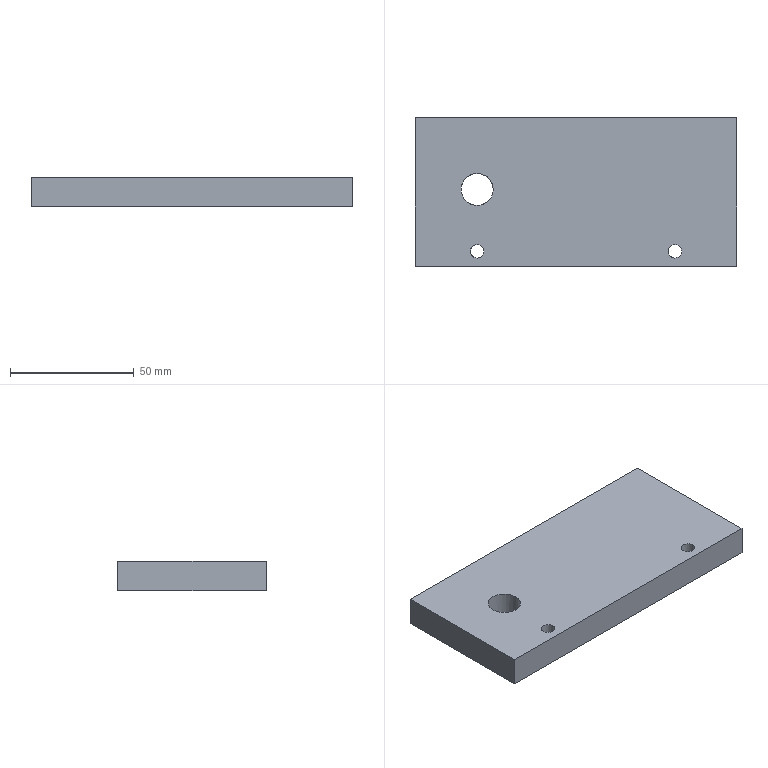Component | NX | Root-owned geometry | 1 solid | 13 faces | box 130 x 60 x 12 mm | volume 90813 mm3 | plane 8 | cylinder 5 | commonest cylinder face diameters 5.5 x2 10 x2 13 x1
STEP:
#1=CARTESIAN_POINT('',(0.,0.,0.));
#2=DIRECTION('',(0.,0.,1.));
#3=DIRECTION('',(1.,0.,0.));
#4=AXIS2_PLACEMENT_3D('',#1,#2,#3);
#5=CARTESIAN_POINT('',(40.,-21.25,12.));
#6=VERTEX_POINT('',#5);
#7=CARTESIAN_POINT('',(40.,-24.,12.));
#8=DIRECTION('',(0.,0.,-1.));
#9=DIRECTION('',(0.,1.,0.));
#10=AXIS2_PLACEMENT_3D('',#7,#8,#9);
#11=CIRCLE('',#10,2.75);
#12=CARTESIAN_POINT('',(40.,-24.,-20.));
#13=DIRECTION('',(0.,0.,1.));
#14=DIRECTION('',(1.,0.,0.));
#15=AXIS2_PLACEMENT_3D('',#12,#13,#14);
#16=CYLINDRICAL_SURFACE('',#15,2.75);
#17=CARTESIAN_POINT('',(7.854,32.));
#18=DIRECTION('',(-1.,0.));
#19=VECTOR('',#18,1.);
#20=LINE('',#17,#19);
#21=(GEOMETRIC_REPRESENTATION_CONTEXT(2)PARAMETRIC_REPRESENTATION_CONTEXT()REPRESENTATION_CONTEXT('',''));
#22=DEFINITIONAL_REPRESENTATION('',(#20),#21);
#23=PCURVE('',#16,#22);
#24=CARTESIAN_POINT('',(0.,0.,12.));
#25=DIRECTION('',(0.,0.,1.));
#26=DIRECTION('',(1.,0.,0.));
#27=AXIS2_PLACEMENT_3D('',#24,#25,#26);
#28=PLANE('',#27);
#29=CARTESIAN_POINT('',(40.,-21.25));
#30=CARTESIAN_POINT('',(44.763,-21.25));
#31=CARTESIAN_POINT('',(42.382,-25.375));
#32=CARTESIAN_POINT('',(40.,-29.5));
#33=CARTESIAN_POINT('',(37.618,-25.375));
#34=CARTESIAN_POINT('',(35.237,-21.25));
#35=CARTESIAN_POINT('',(40.,-21.25));
#36=(BOUNDED_CURVE()B_SPLINE_CURVE(2,(#29,#30,#31,#32,#33,#34,#35),.UNSPECIFIED.,.T.,.F.)B_SPLINE_CURVE_WITH_KNOTS((1,2,2,2,2,1),(-2.094,0.,2.094,4.189,6.283,8.378),.UNSPECIFIED.)CURVE()GEOMETRIC_REPRESENTATION_ITEM()RATIONAL_B_SPLINE_CURVE((1.,0.5,1.,0.5,1.,0.5,1.))REPRESENTATION_ITEM(''));
#37=(GEOMETRIC_REPRESENTATION_CONTEXT(2)PARAMETRIC_REPRESENTATION_CONTEXT()REPRESENTATION_CONTEXT('',''));
#38=DEFINITIONAL_REPRESENTATION('',(#36),#37);
#39=PCURVE('',#28,#38);
#40=SURFACE_CURVE('',#11,(#23,#39),.PCURVE_S1.);
#41=EDGE_CURVE('',#6,#6,#40,.T.);
#42=ORIENTED_EDGE('',*,*,#41,.T.);
#43=CARTESIAN_POINT('',(40.,-21.25,5.7));
#44=VERTEX_POINT('',#43);
#45=CARTESIAN_POINT('',(40.,-21.25,5.7));
#46=CARTESIAN_POINT('',(40.,-21.25,12.));
#47=B_SPLINE_CURVE_WITH_KNOTS('',1,(#45,#46),.UNSPECIFIED.,.F.,.F.,(2,2),(25.7,32.),.PIECEWISE_BEZIER_KNOTS.);
#48=CARTESIAN_POINT('',(1.571,0.));
#49=DIRECTION('',(0.,1.));
#50=VECTOR('',#49,1.);
#51=LINE('',#48,#50);
#52=(GEOMETRIC_REPRESENTATION_CONTEXT(2)PARAMETRIC_REPRESENTATION_CONTEXT()REPRESENTATION_CONTEXT('',''));
#53=DEFINITIONAL_REPRESENTATION('',(#51),#52);
#54=PCURVE('',#16,#53);
#55=CARTESIAN_POINT('',(7.854,0.));
#56=DIRECTION('',(0.,1.));
#57=VECTOR('',#56,1.);
#58=LINE('',#55,#57);
#59=(GEOMETRIC_REPRESENTATION_CONTEXT(2)PARAMETRIC_REPRESENTATION_CONTEXT()REPRESENTATION_CONTEXT('',''));
#60=DEFINITIONAL_REPRESENTATION('',(#58),#59);
#61=PCURVE('',#16,#60);
#62=SEAM_CURVE('',#47,(#54,#61),.PCURVE_S1.);
#63=EDGE_CURVE('',#44,#6,#62,.T.);
#64=ORIENTED_EDGE('',*,*,#63,.F.);
#65=CARTESIAN_POINT('',(37.25,-24.,5.7));
#66=VERTEX_POINT('',#65);
#67=CARTESIAN_POINT('',(40.,-24.,5.7));
#68=DIRECTION('',(0.,0.,-1.));
#69=DIRECTION('',(-1.,0.,0.));
#70=AXIS2_PLACEMENT_3D('',#67,#68,#69);
#71=CIRCLE('',#70,2.75);
#72=CARTESIAN_POINT('',(3.142,25.7));
#73=DIRECTION('',(-1.,0.));
#74=VECTOR('',#73,1.);
#75=LINE('',#72,#74);
#76=(GEOMETRIC_REPRESENTATION_CONTEXT(2)PARAMETRIC_REPRESENTATION_CONTEXT()REPRESENTATION_CONTEXT('',''));
#77=DEFINITIONAL_REPRESENTATION('',(#75),#76);
#78=PCURVE('',#16,#77);
#79=CARTESIAN_POINT('',(40.,-24.,5.7));
#80=DIRECTION('',(0.,0.,-1.));
#81=DIRECTION('',(-1.,0.,0.));
#82=AXIS2_PLACEMENT_3D('',#79,#80,#81);
#83=PLANE('',#82);
#84=CARTESIAN_POINT('',(0.,0.));
#85=DIRECTION('',(1.,0.));
#86=AXIS2_PLACEMENT_2D('',#84,#85);
#87=CIRCLE('',#86,2.75);
#88=(GEOMETRIC_REPRESENTATION_CONTEXT(2)PARAMETRIC_REPRESENTATION_CONTEXT()REPRESENTATION_CONTEXT('',''));
#89=DEFINITIONAL_REPRESENTATION('',(#87),#88);
#90=PCURVE('',#83,#89);
#91=SURFACE_CURVE('',#71,(#78,#90),.PCURVE_S1.);
#92=EDGE_CURVE('',#66,#44,#91,.T.);
#93=ORIENTED_EDGE('',*,*,#92,.F.);
#94=CARTESIAN_POINT('',(40.,-24.,5.7));
#95=DIRECTION('',(0.,0.,-1.));
#96=DIRECTION('',(-1.,0.,0.));
#97=AXIS2_PLACEMENT_3D('',#94,#95,#96);
#98=CIRCLE('',#97,2.75);
#99=CARTESIAN_POINT('',(9.425,25.7));
#100=DIRECTION('',(-1.,0.));
#101=VECTOR('',#100,1.);
#102=LINE('',#99,#101);
#103=(GEOMETRIC_REPRESENTATION_CONTEXT(2)PARAMETRIC_REPRESENTATION_CONTEXT()REPRESENTATION_CONTEXT('',''));
#104=DEFINITIONAL_REPRESENTATION('',(#102),#103);
#105=PCURVE('',#16,#104);
#106=CARTESIAN_POINT('',(0.,0.));
#107=DIRECTION('',(1.,0.));
#108=AXIS2_PLACEMENT_2D('',#106,#107);
#109=CIRCLE('',#108,2.75);
#110=(GEOMETRIC_REPRESENTATION_CONTEXT(2)PARAMETRIC_REPRESENTATION_CONTEXT()REPRESENTATION_CONTEXT('',''));
#111=DEFINITIONAL_REPRESENTATION('',(#109),#110);
#112=PCURVE('',#83,#111);
#113=SURFACE_CURVE('',#98,(#105,#112),.PCURVE_S1.);
#114=EDGE_CURVE('',#44,#66,#113,.T.);
#115=ORIENTED_EDGE('',*,*,#114,.F.);
#116=ORIENTED_EDGE('',*,*,#63,.T.);
#117=EDGE_LOOP('',(#42,#64,#93,#115,#116));
#118=FACE_BOUND('',#117,.F.);
#119=ADVANCED_FACE('',(#118),#16,.F.);
#120=CARTESIAN_POINT('',(-40.,-21.25,12.));
#121=VERTEX_POINT('',#120);
#122=CARTESIAN_POINT('',(-40.,-24.,12.));
#123=DIRECTION('',(0.,0.,-1.));
#124=DIRECTION('',(0.,1.,0.));
#125=AXIS2_PLACEMENT_3D('',#122,#123,#124);
#126=CIRCLE('',#125,2.75);
#127=CARTESIAN_POINT('',(-40.,-24.,-20.));
#128=DIRECTION('',(0.,0.,1.));
#129=DIRECTION('',(1.,0.,0.));
#130=AXIS2_PLACEMENT_3D('',#127,#128,#129);
#131=CYLINDRICAL_SURFACE('',#130,2.75);
#132=CARTESIAN_POINT('',(7.854,32.));
#133=DIRECTION('',(-1.,0.));
#134=VECTOR('',#133,1.);
#135=LINE('',#132,#134);
#136=(GEOMETRIC_REPRESENTATION_CONTEXT(2)PARAMETRIC_REPRESENTATION_CONTEXT()REPRESENTATION_CONTEXT('',''));
#137=DEFINITIONAL_REPRESENTATION('',(#135),#136);
#138=PCURVE('',#131,#137);
#139=CARTESIAN_POINT('',(-40.,-21.25));
#140=CARTESIAN_POINT('',(-35.237,-21.25));
#141=CARTESIAN_POINT('',(-37.618,-25.375));
#142=CARTESIAN_POINT('',(-40.,-29.5));
#143=CARTESIAN_POINT('',(-42.382,-25.375));
#144=CARTESIAN_POINT('',(-44.763,-21.25));
#145=CARTESIAN_POINT('',(-40.,-21.25));
#146=(BOUNDED_CURVE()B_SPLINE_CURVE(2,(#139,#140,#141,#142,#143,#144,#145),.UNSPECIFIED.,.T.,.F.)B_SPLINE_CURVE_WITH_KNOTS((1,2,2,2,2,1),(-2.094,0.,2.094,4.189,6.283,8.378),.UNSPECIFIED.)CURVE()GEOMETRIC_REPRESENTATION_ITEM()RATIONAL_B_SPLINE_CURVE((1.,0.5,1.,0.5,1.,0.5,1.))REPRESENTATION_ITEM(''));
#147=(GEOMETRIC_REPRESENTATION_CONTEXT(2)PARAMETRIC_REPRESENTATION_CONTEXT()REPRESENTATION_CONTEXT('',''));
#148=DEFINITIONAL_REPRESENTATION('',(#146),#147);
#149=PCURVE('',#28,#148);
#150=SURFACE_CURVE('',#126,(#138,#149),.PCURVE_S1.);
#151=EDGE_CURVE('',#121,#121,#150,.T.);
#152=ORIENTED_EDGE('',*,*,#151,.T.);
#153=CARTESIAN_POINT('',(-40.,-21.25,5.7));
#154=VERTEX_POINT('',#153);
#155=CARTESIAN_POINT('',(-40.,-21.25,5.7));
#156=CARTESIAN_POINT('',(-40.,-21.25,12.));
#157=B_SPLINE_CURVE_WITH_KNOTS('',1,(#155,#156),.UNSPECIFIED.,.F.,.F.,(2,2),(25.7,32.),.PIECEWISE_BEZIER_KNOTS.);
#158=CARTESIAN_POINT('',(1.571,0.));
#159=DIRECTION('',(0.,1.));
#160=VECTOR('',#159,1.);
#161=LINE('',#158,#160);
#162=(GEOMETRIC_REPRESENTATION_CONTEXT(2)PARAMETRIC_REPRESENTATION_CONTEXT()REPRESENTATION_CONTEXT('',''));
#163=DEFINITIONAL_REPRESENTATION('',(#161),#162);
#164=PCURVE('',#131,#163);
#165=CARTESIAN_POINT('',(7.854,0.));
#166=DIRECTION('',(0.,1.));
#167=VECTOR('',#166,1.);
#168=LINE('',#165,#167);
#169=(GEOMETRIC_REPRESENTATION_CONTEXT(2)PARAMETRIC_REPRESENTATION_CONTEXT()REPRESENTATION_CONTEXT('',''));
#170=DEFINITIONAL_REPRESENTATION('',(#168),#169);
#171=PCURVE('',#131,#170);
#172=SEAM_CURVE('',#157,(#164,#171),.PCURVE_S1.);
#173=EDGE_CURVE('',#154,#121,#172,.T.);
#174=ORIENTED_EDGE('',*,*,#173,.F.);
#175=CARTESIAN_POINT('',(-42.75,-24.,5.7));
#176=VERTEX_POINT('',#175);
#177=CARTESIAN_POINT('',(-40.,-24.,5.7));
#178=DIRECTION('',(0.,0.,-1.));
#179=DIRECTION('',(-1.,0.,0.));
#180=AXIS2_PLACEMENT_3D('',#177,#178,#179);
#181=CIRCLE('',#180,2.75);
#182=CARTESIAN_POINT('',(3.142,25.7));
#183=DIRECTION('',(-1.,0.));
#184=VECTOR('',#183,1.);
#185=LINE('',#182,#184);
#186=(GEOMETRIC_REPRESENTATION_CONTEXT(2)PARAMETRIC_REPRESENTATION_CONTEXT()REPRESENTATION_CONTEXT('',''));
#187=DEFINITIONAL_REPRESENTATION('',(#185),#186);
#188=PCURVE('',#131,#187);
#189=CARTESIAN_POINT('',(-40.,-24.,5.7));
#190=DIRECTION('',(0.,0.,-1.));
#191=DIRECTION('',(-1.,0.,0.));
#192=AXIS2_PLACEMENT_3D('',#189,#190,#191);
#193=PLANE('',#192);
#194=CARTESIAN_POINT('',(0.,0.));
#195=DIRECTION('',(1.,0.));
#196=AXIS2_PLACEMENT_2D('',#194,#195);
#197=CIRCLE('',#196,2.75);
#198=(GEOMETRIC_REPRESENTATION_CONTEXT(2)PARAMETRIC_REPRESENTATION_CONTEXT()REPRESENTATION_CONTEXT('',''));
#199=DEFINITIONAL_REPRESENTATION('',(#197),#198);
#200=PCURVE('',#193,#199);
#201=SURFACE_CURVE('',#181,(#188,#200),.PCURVE_S1.);
#202=EDGE_CURVE('',#176,#154,#201,.T.);
#203=ORIENTED_EDGE('',*,*,#202,.F.);
#204=CARTESIAN_POINT('',(-40.,-24.,5.7));
#205=DIRECTION('',(0.,0.,-1.));
#206=DIRECTION('',(-1.,0.,0.));
#207=AXIS2_PLACEMENT_3D('',#204,#205,#206);
#208=CIRCLE('',#207,2.75);
#209=CARTESIAN_POINT('',(9.425,25.7));
#210=DIRECTION('',(-1.,0.));
#211=VECTOR('',#210,1.);
#212=LINE('',#209,#211);
#213=(GEOMETRIC_REPRESENTATION_CONTEXT(2)PARAMETRIC_REPRESENTATION_CONTEXT()REPRESENTATION_CONTEXT('',''));
#214=DEFINITIONAL_REPRESENTATION('',(#212),#213);
#215=PCURVE('',#131,#214);
#216=CARTESIAN_POINT('',(0.,0.));
#217=DIRECTION('',(1.,0.));
#218=AXIS2_PLACEMENT_2D('',#216,#217);
#219=CIRCLE('',#218,2.75);
#220=(GEOMETRIC_REPRESENTATION_CONTEXT(2)PARAMETRIC_REPRESENTATION_CONTEXT()REPRESENTATION_CONTEXT('',''));
#221=DEFINITIONAL_REPRESENTATION('',(#219),#220);
#222=PCURVE('',#193,#221);
#223=SURFACE_CURVE('',#208,(#215,#222),.PCURVE_S1.);
#224=EDGE_CURVE('',#154,#176,#223,.T.);
#225=ORIENTED_EDGE('',*,*,#224,.F.);
#226=ORIENTED_EDGE('',*,*,#173,.T.);
#227=EDGE_LOOP('',(#152,#174,#203,#225,#226));
#228=FACE_BOUND('',#227,.F.);
#229=ADVANCED_FACE('',(#228),#131,.F.);
#230=CARTESIAN_POINT('',(-65.,-30.,0.));
#231=VERTEX_POINT('',#230);
#232=CARTESIAN_POINT('',(65.,-30.,0.));
#233=VERTEX_POINT('',#232);
#234=CARTESIAN_POINT('',(-65.,-30.,0.));
#235=DIRECTION('',(1.,0.,0.));
#236=VECTOR('',#235,1.);
#237=LINE('',#234,#236);
#238=CARTESIAN_POINT('',(-65.,-30.,12.));
#239=DIRECTION('',(-0.,1.,0.));
#240=DIRECTION('',(-1.,-0.,0.));
#241=AXIS2_PLACEMENT_3D('',#238,#239,#240);
#242=PLANE('',#241);
#243=CARTESIAN_POINT('',(0.,-12.));
#244=DIRECTION('',(-1.,0.));
#245=VECTOR('',#244,1.);
#246=LINE('',#243,#245);
#247=(GEOMETRIC_REPRESENTATION_CONTEXT(2)PARAMETRIC_REPRESENTATION_CONTEXT()REPRESENTATION_CONTEXT('',''));
#248=DEFINITIONAL_REPRESENTATION('',(#246),#247);
#249=PCURVE('',#242,#248);
#250=CARTESIAN_POINT('',(0.,0.,0.));
#251=DIRECTION('',(0.,0.,1.));
#252=DIRECTION('',(1.,0.,0.));
#253=AXIS2_PLACEMENT_3D('',#250,#251,#252);
#254=PLANE('',#253);
#255=CARTESIAN_POINT('',(-65.,-30.));
#256=DIRECTION('',(1.,0.));
#257=VECTOR('',#256,1.);
#258=LINE('',#255,#257);
#259=(GEOMETRIC_REPRESENTATION_CONTEXT(2)PARAMETRIC_REPRESENTATION_CONTEXT()REPRESENTATION_CONTEXT('',''));
#260=DEFINITIONAL_REPRESENTATION('',(#258),#259);
#261=PCURVE('',#254,#260);
#262=SURFACE_CURVE('',#237,(#249,#261),.PCURVE_S1.);
#263=EDGE_CURVE('',#231,#233,#262,.T.);
#264=ORIENTED_EDGE('',*,*,#263,.T.);
#265=CARTESIAN_POINT('',(65.,-30.,12.));
#266=VERTEX_POINT('',#265);
#267=CARTESIAN_POINT('',(65.,-30.,12.));
#268=DIRECTION('',(0.,0.,-1.));
#269=VECTOR('',#268,1.);
#270=LINE('',#267,#269);
#271=CARTESIAN_POINT('',(-130.,0.));
#272=DIRECTION('',(0.,-1.));
#273=VECTOR('',#272,1.);
#274=LINE('',#271,#273);
#275=(GEOMETRIC_REPRESENTATION_CONTEXT(2)PARAMETRIC_REPRESENTATION_CONTEXT()REPRESENTATION_CONTEXT('',''));
#276=DEFINITIONAL_REPRESENTATION('',(#274),#275);
#277=PCURVE('',#242,#276);
#278=CARTESIAN_POINT('',(65.,-30.,12.));
#279=DIRECTION('',(-1.,-0.,0.));
#280=DIRECTION('',(0.,-1.,0.));
#281=AXIS2_PLACEMENT_3D('',#278,#279,#280);
#282=PLANE('',#281);
#283=CARTESIAN_POINT('',(0.,0.));
#284=DIRECTION('',(0.,-1.));
#285=VECTOR('',#284,1.);
#286=LINE('',#283,#285);
#287=(GEOMETRIC_REPRESENTATION_CONTEXT(2)PARAMETRIC_REPRESENTATION_CONTEXT()REPRESENTATION_CONTEXT('',''));
#288=DEFINITIONAL_REPRESENTATION('',(#286),#287);
#289=PCURVE('',#282,#288);
#290=SURFACE_CURVE('',#270,(#277,#289),.PCURVE_S1.);
#291=EDGE_CURVE('',#266,#233,#290,.T.);
#292=ORIENTED_EDGE('',*,*,#291,.F.);
#293=CARTESIAN_POINT('',(-65.,-30.,12.));
#294=VERTEX_POINT('',#293);
#295=CARTESIAN_POINT('',(-65.,-30.,12.));
#296=DIRECTION('',(1.,0.,0.));
#297=VECTOR('',#296,1.);
#298=LINE('',#295,#297);
#299=CARTESIAN_POINT('',(0.,0.));
#300=DIRECTION('',(-1.,0.));
#301=VECTOR('',#300,1.);
#302=LINE('',#299,#301);
#303=(GEOMETRIC_REPRESENTATION_CONTEXT(2)PARAMETRIC_REPRESENTATION_CONTEXT()REPRESENTATION_CONTEXT('',''));
#304=DEFINITIONAL_REPRESENTATION('',(#302),#303);
#305=PCURVE('',#242,#304);
#306=CARTESIAN_POINT('',(-65.,-30.));
#307=DIRECTION('',(1.,0.));
#308=VECTOR('',#307,1.);
#309=LINE('',#306,#308);
#310=(GEOMETRIC_REPRESENTATION_CONTEXT(2)PARAMETRIC_REPRESENTATION_CONTEXT()REPRESENTATION_CONTEXT('',''));
#311=DEFINITIONAL_REPRESENTATION('',(#309),#310);
#312=PCURVE('',#28,#311);
#313=SURFACE_CURVE('',#298,(#305,#312),.PCURVE_S1.);
#314=EDGE_CURVE('',#294,#266,#313,.T.);
#315=ORIENTED_EDGE('',*,*,#314,.F.);
#316=CARTESIAN_POINT('',(-65.,-30.,12.));
#317=DIRECTION('',(0.,0.,-1.));
#318=VECTOR('',#317,1.);
#319=LINE('',#316,#318);
#320=CARTESIAN_POINT('',(0.,0.));
#321=DIRECTION('',(0.,-1.));
#322=VECTOR('',#321,1.);
#323=LINE('',#320,#322);
#324=(GEOMETRIC_REPRESENTATION_CONTEXT(2)PARAMETRIC_REPRESENTATION_CONTEXT()REPRESENTATION_CONTEXT('',''));
#325=DEFINITIONAL_REPRESENTATION('',(#323),#324);
#326=PCURVE('',#242,#325);
#327=CARTESIAN_POINT('',(-65.,30.,12.));
#328=DIRECTION('',(1.,0.,0.));
#329=DIRECTION('',(0.,0.,-1.));
#330=AXIS2_PLACEMENT_3D('',#327,#328,#329);
#331=PLANE('',#330);
#332=CARTESIAN_POINT('',(0.,-60.));
#333=DIRECTION('',(1.,0.));
#334=VECTOR('',#333,1.);
#335=LINE('',#332,#334);
#336=(GEOMETRIC_REPRESENTATION_CONTEXT(2)PARAMETRIC_REPRESENTATION_CONTEXT()REPRESENTATION_CONTEXT('',''));
#337=DEFINITIONAL_REPRESENTATION('',(#335),#336);
#338=PCURVE('',#331,#337);
#339=SURFACE_CURVE('',#319,(#326,#338),.PCURVE_S1.);
#340=EDGE_CURVE('',#294,#231,#339,.T.);
#341=ORIENTED_EDGE('',*,*,#340,.T.);
#342=EDGE_LOOP('',(#264,#292,#315,#341));
#343=FACE_BOUND('',#342,.T.);
#344=ADVANCED_FACE('',(#343),#242,.F.);
#345=CARTESIAN_POINT('',(65.,30.,0.));
#346=VERTEX_POINT('',#345);
#347=CARTESIAN_POINT('',(65.,-30.,0.));
#348=DIRECTION('',(-0.,1.,0.));
#349=VECTOR('',#348,1.);
#350=LINE('',#347,#349);
#351=CARTESIAN_POINT('',(0.,-12.));
#352=DIRECTION('',(-1.,0.));
#353=VECTOR('',#352,1.);
#354=LINE('',#351,#353);
#355=(GEOMETRIC_REPRESENTATION_CONTEXT(2)PARAMETRIC_REPRESENTATION_CONTEXT()REPRESENTATION_CONTEXT('',''));
#356=DEFINITIONAL_REPRESENTATION('',(#354),#355);
#357=PCURVE('',#282,#356);
#358=CARTESIAN_POINT('',(65.,-30.));
#359=DIRECTION('',(-0.,1.));
#360=VECTOR('',#359,1.);
#361=LINE('',#358,#360);
#362=(GEOMETRIC_REPRESENTATION_CONTEXT(2)PARAMETRIC_REPRESENTATION_CONTEXT()REPRESENTATION_CONTEXT('',''));
#363=DEFINITIONAL_REPRESENTATION('',(#361),#362);
#364=PCURVE('',#254,#363);
#365=SURFACE_CURVE('',#350,(#357,#364),.PCURVE_S1.);
#366=EDGE_CURVE('',#233,#346,#365,.T.);
#367=ORIENTED_EDGE('',*,*,#366,.T.);
#368=CARTESIAN_POINT('',(65.,30.,12.));
#369=VERTEX_POINT('',#368);
#370=CARTESIAN_POINT('',(65.,30.,12.));
#371=DIRECTION('',(0.,0.,-1.));
#372=VECTOR('',#371,1.);
#373=LINE('',#370,#372);
#374=CARTESIAN_POINT('',(-60.,0.));
#375=DIRECTION('',(0.,-1.));
#376=VECTOR('',#375,1.);
#377=LINE('',#374,#376);
#378=(GEOMETRIC_REPRESENTATION_CONTEXT(2)PARAMETRIC_REPRESENTATION_CONTEXT()REPRESENTATION_CONTEXT('',''));
#379=DEFINITIONAL_REPRESENTATION('',(#377),#378);
#380=PCURVE('',#282,#379);
#381=CARTESIAN_POINT('',(65.,30.,12.));
#382=DIRECTION('',(0.,-1.,0.));
#383=DIRECTION('',(0.,0.,-1.));
#384=AXIS2_PLACEMENT_3D('',#381,#382,#383);
#385=PLANE('',#384);
#386=CARTESIAN_POINT('',(0.,0.));
#387=DIRECTION('',(1.,0.));
#388=VECTOR('',#387,1.);
#389=LINE('',#386,#388);
#390=(GEOMETRIC_REPRESENTATION_CONTEXT(2)PARAMETRIC_REPRESENTATION_CONTEXT()REPRESENTATION_CONTEXT('',''));
#391=DEFINITIONAL_REPRESENTATION('',(#389),#390);
#392=PCURVE('',#385,#391);
#393=SURFACE_CURVE('',#373,(#380,#392),.PCURVE_S1.);
#394=EDGE_CURVE('',#369,#346,#393,.T.);
#395=ORIENTED_EDGE('',*,*,#394,.F.);
#396=CARTESIAN_POINT('',(65.,-30.,12.));
#397=DIRECTION('',(-0.,1.,0.));
#398=VECTOR('',#397,1.);
#399=LINE('',#396,#398);
#400=CARTESIAN_POINT('',(0.,0.));
#401=DIRECTION('',(-1.,0.));
#402=VECTOR('',#401,1.);
#403=LINE('',#400,#402);
#404=(GEOMETRIC_REPRESENTATION_CONTEXT(2)PARAMETRIC_REPRESENTATION_CONTEXT()REPRESENTATION_CONTEXT('',''));
#405=DEFINITIONAL_REPRESENTATION('',(#403),#404);
#406=PCURVE('',#282,#405);
#407=CARTESIAN_POINT('',(65.,-30.));
#408=DIRECTION('',(-0.,1.));
#409=VECTOR('',#408,1.);
#410=LINE('',#407,#409);
#411=(GEOMETRIC_REPRESENTATION_CONTEXT(2)PARAMETRIC_REPRESENTATION_CONTEXT()REPRESENTATION_CONTEXT('',''));
#412=DEFINITIONAL_REPRESENTATION('',(#410),#411);
#413=PCURVE('',#28,#412);
#414=SURFACE_CURVE('',#399,(#406,#413),.PCURVE_S1.);
#415=EDGE_CURVE('',#266,#369,#414,.T.);
#416=ORIENTED_EDGE('',*,*,#415,.F.);
#417=ORIENTED_EDGE('',*,*,#291,.T.);
#418=EDGE_LOOP('',(#367,#395,#416,#417));
#419=FACE_BOUND('',#418,.T.);
#420=ADVANCED_FACE('',(#419),#282,.F.);
#421=CARTESIAN_POINT('',(-65.,30.,0.));
#422=VERTEX_POINT('',#421);
#423=CARTESIAN_POINT('',(65.,30.,0.));
#424=DIRECTION('',(-1.,0.,0.));
#425=VECTOR('',#424,1.);
#426=LINE('',#423,#425);
#427=CARTESIAN_POINT('',(12.,0.));
#428=DIRECTION('',(0.,-1.));
#429=VECTOR('',#428,1.);
#430=LINE('',#427,#429);
#431=(GEOMETRIC_REPRESENTATION_CONTEXT(2)PARAMETRIC_REPRESENTATION_CONTEXT()REPRESENTATION_CONTEXT('',''));
#432=DEFINITIONAL_REPRESENTATION('',(#430),#431);
#433=PCURVE('',#385,#432);
#434=CARTESIAN_POINT('',(65.,30.));
#435=DIRECTION('',(-1.,0.));
#436=VECTOR('',#435,1.);
#437=LINE('',#434,#436);
#438=(GEOMETRIC_REPRESENTATION_CONTEXT(2)PARAMETRIC_REPRESENTATION_CONTEXT()REPRESENTATION_CONTEXT('',''));
#439=DEFINITIONAL_REPRESENTATION('',(#437),#438);
#440=PCURVE('',#254,#439);
#441=SURFACE_CURVE('',#426,(#433,#440),.PCURVE_S1.);
#442=EDGE_CURVE('',#346,#422,#441,.T.);
#443=ORIENTED_EDGE('',*,*,#442,.T.);
#444=CARTESIAN_POINT('',(-65.,30.,12.));
#445=VERTEX_POINT('',#444);
#446=CARTESIAN_POINT('',(-65.,30.,12.));
#447=DIRECTION('',(0.,0.,-1.));
#448=VECTOR('',#447,1.);
#449=LINE('',#446,#448);
#450=CARTESIAN_POINT('',(0.,-130.));
#451=DIRECTION('',(1.,0.));
#452=VECTOR('',#451,1.);
#453=LINE('',#450,#452);
#454=(GEOMETRIC_REPRESENTATION_CONTEXT(2)PARAMETRIC_REPRESENTATION_CONTEXT()REPRESENTATION_CONTEXT('',''));
#455=DEFINITIONAL_REPRESENTATION('',(#453),#454);
#456=PCURVE('',#385,#455);
#457=CARTESIAN_POINT('',(0.,0.));
#458=DIRECTION('',(1.,0.));
#459=VECTOR('',#458,1.);
#460=LINE('',#457,#459);
#461=(GEOMETRIC_REPRESENTATION_CONTEXT(2)PARAMETRIC_REPRESENTATION_CONTEXT()REPRESENTATION_CONTEXT('',''));
#462=DEFINITIONAL_REPRESENTATION('',(#460),#461);
#463=PCURVE('',#331,#462);
#464=SURFACE_CURVE('',#449,(#456,#463),.PCURVE_S1.);
#465=EDGE_CURVE('',#445,#422,#464,.T.);
#466=ORIENTED_EDGE('',*,*,#465,.F.);
#467=CARTESIAN_POINT('',(65.,30.,12.));
#468=DIRECTION('',(-1.,0.,0.));
#469=VECTOR('',#468,1.);
#470=LINE('',#467,#469);
#471=CARTESIAN_POINT('',(0.,0.));
#472=DIRECTION('',(0.,-1.));
#473=VECTOR('',#472,1.);
#474=LINE('',#471,#473);
#475=(GEOMETRIC_REPRESENTATION_CONTEXT(2)PARAMETRIC_REPRESENTATION_CONTEXT()REPRESENTATION_CONTEXT('',''));
#476=DEFINITIONAL_REPRESENTATION('',(#474),#475);
#477=PCURVE('',#385,#476);
#478=CARTESIAN_POINT('',(65.,30.));
#479=DIRECTION('',(-1.,0.));
#480=VECTOR('',#479,1.);
#481=LINE('',#478,#480);
#482=(GEOMETRIC_REPRESENTATION_CONTEXT(2)PARAMETRIC_REPRESENTATION_CONTEXT()REPRESENTATION_CONTEXT('',''));
#483=DEFINITIONAL_REPRESENTATION('',(#481),#482);
#484=PCURVE('',#28,#483);
#485=SURFACE_CURVE('',#470,(#477,#484),.PCURVE_S1.);
#486=EDGE_CURVE('',#369,#445,#485,.T.);
#487=ORIENTED_EDGE('',*,*,#486,.F.);
#488=ORIENTED_EDGE('',*,*,#394,.T.);
#489=EDGE_LOOP('',(#443,#466,#487,#488));
#490=FACE_BOUND('',#489,.T.);
#491=ADVANCED_FACE('',(#490),#385,.F.);
#492=CARTESIAN_POINT('',(-65.,30.,0.));
#493=DIRECTION('',(0.,-1.,0.));
#494=VECTOR('',#493,1.);
#495=LINE('',#492,#494);
#496=CARTESIAN_POINT('',(12.,0.));
#497=DIRECTION('',(0.,-1.));
#498=VECTOR('',#497,1.);
#499=LINE('',#496,#498);
#500=(GEOMETRIC_REPRESENTATION_CONTEXT(2)PARAMETRIC_REPRESENTATION_CONTEXT()REPRESENTATION_CONTEXT('',''));
#501=DEFINITIONAL_REPRESENTATION('',(#499),#500);
#502=PCURVE('',#331,#501);
#503=CARTESIAN_POINT('',(-65.,30.));
#504=DIRECTION('',(0.,-1.));
#505=VECTOR('',#504,1.);
#506=LINE('',#503,#505);
#507=(GEOMETRIC_REPRESENTATION_CONTEXT(2)PARAMETRIC_REPRESENTATION_CONTEXT()REPRESENTATION_CONTEXT('',''));
#508=DEFINITIONAL_REPRESENTATION('',(#506),#507);
#509=PCURVE('',#254,#508);
#510=SURFACE_CURVE('',#495,(#502,#509),.PCURVE_S1.);
#511=EDGE_CURVE('',#422,#231,#510,.T.);
#512=ORIENTED_EDGE('',*,*,#511,.T.);
#513=ORIENTED_EDGE('',*,*,#340,.F.);
#514=CARTESIAN_POINT('',(-65.,30.,12.));
#515=DIRECTION('',(0.,-1.,0.));
#516=VECTOR('',#515,1.);
#517=LINE('',#514,#516);
#518=CARTESIAN_POINT('',(0.,0.));
#519=DIRECTION('',(0.,-1.));
#520=VECTOR('',#519,1.);
#521=LINE('',#518,#520);
#522=(GEOMETRIC_REPRESENTATION_CONTEXT(2)PARAMETRIC_REPRESENTATION_CONTEXT()REPRESENTATION_CONTEXT('',''));
#523=DEFINITIONAL_REPRESENTATION('',(#521),#522);
#524=PCURVE('',#331,#523);
#525=CARTESIAN_POINT('',(-65.,30.));
#526=DIRECTION('',(0.,-1.));
#527=VECTOR('',#526,1.);
#528=LINE('',#525,#527);
#529=(GEOMETRIC_REPRESENTATION_CONTEXT(2)PARAMETRIC_REPRESENTATION_CONTEXT()REPRESENTATION_CONTEXT('',''));
#530=DEFINITIONAL_REPRESENTATION('',(#528),#529);
#531=PCURVE('',#28,#530);
#532=SURFACE_CURVE('',#517,(#524,#531),.PCURVE_S1.);
#533=EDGE_CURVE('',#445,#294,#532,.T.);
#534=ORIENTED_EDGE('',*,*,#533,.F.);
#535=ORIENTED_EDGE('',*,*,#465,.T.);
#536=EDGE_LOOP('',(#512,#513,#534,#535));
#537=FACE_BOUND('',#536,.T.);
#538=ADVANCED_FACE('',(#537),#331,.F.);
#539=ORIENTED_EDGE('',*,*,#41,.T.);
#540=EDGE_LOOP('',(#539));
#541=FACE_BOUND('',#540,.T.);
#542=CARTESIAN_POINT('',(-40.,7.5,12.));
#543=VERTEX_POINT('',#542);
#544=CARTESIAN_POINT('',(-33.5,1.,12.));
#545=VERTEX_POINT('',#544);
#546=CARTESIAN_POINT('',(-40.,1.,12.));
#547=DIRECTION('',(0.,0.,-1.));
#548=DIRECTION('',(0.,1.,0.));
#549=AXIS2_PLACEMENT_3D('',#546,#547,#548);
#550=CIRCLE('',#549,6.5);
#551=CARTESIAN_POINT('',(-40.,7.5));
#552=CARTESIAN_POINT('',(-28.742,7.5));
#553=CARTESIAN_POINT('',(-34.371,-2.25));
#554=CARTESIAN_POINT('',(-40.,-12.));
#555=CARTESIAN_POINT('',(-45.629,-2.25));
#556=CARTESIAN_POINT('',(-51.258,7.5));
#557=CARTESIAN_POINT('',(-40.,7.5));
#558=(BOUNDED_CURVE()B_SPLINE_CURVE(2,(#551,#552,#553,#554,#555,#556,#557),.UNSPECIFIED.,.T.,.F.)B_SPLINE_CURVE_WITH_KNOTS((1,2,2,2,2,1),(-2.094,0.,2.094,4.189,6.283,8.378),.UNSPECIFIED.)CURVE()GEOMETRIC_REPRESENTATION_ITEM()RATIONAL_B_SPLINE_CURVE((1.,0.5,1.,0.5,1.,0.5,1.))REPRESENTATION_ITEM(''));
#559=(GEOMETRIC_REPRESENTATION_CONTEXT(2)PARAMETRIC_REPRESENTATION_CONTEXT()REPRESENTATION_CONTEXT('',''));
#560=DEFINITIONAL_REPRESENTATION('',(#558),#559);
#561=PCURVE('',#28,#560);
#562=CARTESIAN_POINT('',(-40.,1.,-20.));
#563=DIRECTION('',(0.,0.,1.));
#564=DIRECTION('',(1.,0.,0.));
#565=AXIS2_PLACEMENT_3D('',#562,#563,#564);
#566=CYLINDRICAL_SURFACE('',#565,6.5);
#567=CARTESIAN_POINT('',(1.571,32.));
#568=DIRECTION('',(-1.,0.));
#569=VECTOR('',#568,1.);
#570=LINE('',#567,#569);
#571=(GEOMETRIC_REPRESENTATION_CONTEXT(2)PARAMETRIC_REPRESENTATION_CONTEXT()REPRESENTATION_CONTEXT('',''));
#572=DEFINITIONAL_REPRESENTATION('',(#570),#571);
#573=PCURVE('',#566,#572);
#574=SURFACE_CURVE('',#550,(#561,#573),.PCURVE_S1.);
#575=EDGE_CURVE('',#543,#545,#574,.T.);
#576=ORIENTED_EDGE('',*,*,#575,.T.);
#577=CARTESIAN_POINT('',(-40.,1.,12.));
#578=DIRECTION('',(0.,0.,-1.));
#579=DIRECTION('',(0.,1.,0.));
#580=AXIS2_PLACEMENT_3D('',#577,#578,#579);
#581=CIRCLE('',#580,6.5);
#582=CARTESIAN_POINT('',(-40.,7.5));
#583=CARTESIAN_POINT('',(-28.742,7.5));
#584=CARTESIAN_POINT('',(-34.371,-2.25));
#585=CARTESIAN_POINT('',(-40.,-12.));
#586=CARTESIAN_POINT('',(-45.629,-2.25));
#587=CARTESIAN_POINT('',(-51.258,7.5));
#588=CARTESIAN_POINT('',(-40.,7.5));
#589=(BOUNDED_CURVE()B_SPLINE_CURVE(2,(#582,#583,#584,#585,#586,#587,#588),.UNSPECIFIED.,.T.,.F.)B_SPLINE_CURVE_WITH_KNOTS((1,2,2,2,2,1),(-2.094,0.,2.094,4.189,6.283,8.378),.UNSPECIFIED.)CURVE()GEOMETRIC_REPRESENTATION_ITEM()RATIONAL_B_SPLINE_CURVE((1.,0.5,1.,0.5,1.,0.5,1.))REPRESENTATION_ITEM(''));
#590=(GEOMETRIC_REPRESENTATION_CONTEXT(2)PARAMETRIC_REPRESENTATION_CONTEXT()REPRESENTATION_CONTEXT('',''));
#591=DEFINITIONAL_REPRESENTATION('',(#589),#590);
#592=PCURVE('',#28,#591);
#593=CARTESIAN_POINT('',(7.854,32.));
#594=DIRECTION('',(-1.,0.));
#595=VECTOR('',#594,1.);
#596=LINE('',#593,#595);
#597=(GEOMETRIC_REPRESENTATION_CONTEXT(2)PARAMETRIC_REPRESENTATION_CONTEXT()REPRESENTATION_CONTEXT('',''));
#598=DEFINITIONAL_REPRESENTATION('',(#596),#597);
#599=PCURVE('',#566,#598);
#600=SURFACE_CURVE('',#581,(#592,#599),.PCURVE_S1.);
#601=EDGE_CURVE('',#545,#543,#600,.T.);
#602=ORIENTED_EDGE('',*,*,#601,.T.);
#603=EDGE_LOOP('',(#576,#602));
#604=FACE_BOUND('',#603,.T.);
#605=ORIENTED_EDGE('',*,*,#151,.T.);
#606=EDGE_LOOP('',(#605));
#607=FACE_BOUND('',#606,.T.);
#608=ORIENTED_EDGE('',*,*,#314,.T.);
#609=ORIENTED_EDGE('',*,*,#415,.T.);
#610=ORIENTED_EDGE('',*,*,#486,.T.);
#611=ORIENTED_EDGE('',*,*,#533,.T.);
#612=EDGE_LOOP('',(#608,#609,#610,#611));
#613=FACE_BOUND('',#612,.T.);
#614=ADVANCED_FACE('',(#541,#604,#607,#613),#28,.T.);
#615=CARTESIAN_POINT('',(45.,-24.,0.));
#616=VERTEX_POINT('',#615);
#617=CARTESIAN_POINT('',(40.,-24.,0.));
#618=DIRECTION('',(0.,0.,-1.));
#619=DIRECTION('',(1.,0.,0.));
#620=AXIS2_PLACEMENT_3D('',#617,#618,#619);
#621=CIRCLE('',#620,5.);
#622=CARTESIAN_POINT('',(45.,-24.));
#623=CARTESIAN_POINT('',(45.,-32.66));
#624=CARTESIAN_POINT('',(37.5,-28.33));
#625=CARTESIAN_POINT('',(30.,-24.));
#626=CARTESIAN_POINT('',(37.5,-19.67));
#627=CARTESIAN_POINT('',(45.,-15.34));
#628=CARTESIAN_POINT('',(45.,-24.));
#629=(BOUNDED_CURVE()B_SPLINE_CURVE(2,(#622,#623,#624,#625,#626,#627,#628),.UNSPECIFIED.,.T.,.F.)B_SPLINE_CURVE_WITH_KNOTS((1,2,2,2,2,1),(-2.094,0.,2.094,4.189,6.283,8.378),.UNSPECIFIED.)CURVE()GEOMETRIC_REPRESENTATION_ITEM()RATIONAL_B_SPLINE_CURVE((1.,0.5,1.,0.5,1.,0.5,1.))REPRESENTATION_ITEM(''));
#630=(GEOMETRIC_REPRESENTATION_CONTEXT(2)PARAMETRIC_REPRESENTATION_CONTEXT()REPRESENTATION_CONTEXT('',''));
#631=DEFINITIONAL_REPRESENTATION('',(#629),#630);
#632=PCURVE('',#254,#631);
#633=CARTESIAN_POINT('',(40.,-24.,5.7));
#634=DIRECTION('',(0.,0.,-1.));
#635=DIRECTION('',(-1.,0.,0.));
#636=AXIS2_PLACEMENT_3D('',#633,#634,#635);
#637=CYLINDRICAL_SURFACE('',#636,5.);
#638=CARTESIAN_POINT('',(3.142,5.7));
#639=DIRECTION('',(1.,0.));
#640=VECTOR('',#639,1.);
#641=LINE('',#638,#640);
#642=(GEOMETRIC_REPRESENTATION_CONTEXT(2)PARAMETRIC_REPRESENTATION_CONTEXT()REPRESENTATION_CONTEXT('',''));
#643=DEFINITIONAL_REPRESENTATION('',(#641),#642);
#644=PCURVE('',#637,#643);
#645=SURFACE_CURVE('',#621,(#632,#644),.PCURVE_S1.);
#646=EDGE_CURVE('',#616,#616,#645,.T.);
#647=ORIENTED_EDGE('',*,*,#646,.F.);
#648=EDGE_LOOP('',(#647));
#649=FACE_BOUND('',#648,.T.);
#650=CARTESIAN_POINT('',(-35.,-24.,0.));
#651=VERTEX_POINT('',#650);
#652=CARTESIAN_POINT('',(-40.,-24.,0.));
#653=DIRECTION('',(0.,0.,-1.));
#654=DIRECTION('',(1.,0.,0.));
#655=AXIS2_PLACEMENT_3D('',#652,#653,#654);
#656=CIRCLE('',#655,5.);
#657=CARTESIAN_POINT('',(-35.,-24.));
#658=CARTESIAN_POINT('',(-35.,-32.66));
#659=CARTESIAN_POINT('',(-42.5,-28.33));
#660=CARTESIAN_POINT('',(-50.,-24.));
#661=CARTESIAN_POINT('',(-42.5,-19.67));
#662=CARTESIAN_POINT('',(-35.,-15.34));
#663=CARTESIAN_POINT('',(-35.,-24.));
#664=(BOUNDED_CURVE()B_SPLINE_CURVE(2,(#657,#658,#659,#660,#661,#662,#663),.UNSPECIFIED.,.T.,.F.)B_SPLINE_CURVE_WITH_KNOTS((1,2,2,2,2,1),(-2.094,0.,2.094,4.189,6.283,8.378),.UNSPECIFIED.)CURVE()GEOMETRIC_REPRESENTATION_ITEM()RATIONAL_B_SPLINE_CURVE((1.,0.5,1.,0.5,1.,0.5,1.))REPRESENTATION_ITEM(''));
#665=(GEOMETRIC_REPRESENTATION_CONTEXT(2)PARAMETRIC_REPRESENTATION_CONTEXT()REPRESENTATION_CONTEXT('',''));
#666=DEFINITIONAL_REPRESENTATION('',(#664),#665);
#667=PCURVE('',#254,#666);
#668=CARTESIAN_POINT('',(-40.,-24.,5.7));
#669=DIRECTION('',(0.,0.,-1.));
#670=DIRECTION('',(-1.,0.,0.));
#671=AXIS2_PLACEMENT_3D('',#668,#669,#670);
#672=CYLINDRICAL_SURFACE('',#671,5.);
#673=CARTESIAN_POINT('',(3.142,5.7));
#674=DIRECTION('',(1.,0.));
#675=VECTOR('',#674,1.);
#676=LINE('',#673,#675);
#677=(GEOMETRIC_REPRESENTATION_CONTEXT(2)PARAMETRIC_REPRESENTATION_CONTEXT()REPRESENTATION_CONTEXT('',''));
#678=DEFINITIONAL_REPRESENTATION('',(#676),#677);
#679=PCURVE('',#672,#678);
#680=SURFACE_CURVE('',#656,(#667,#679),.PCURVE_S1.);
#681=EDGE_CURVE('',#651,#651,#680,.T.);
#682=ORIENTED_EDGE('',*,*,#681,.F.);
#683=EDGE_LOOP('',(#682));
#684=FACE_BOUND('',#683,.T.);
#685=CARTESIAN_POINT('',(-33.5,1.,0.));
#686=VERTEX_POINT('',#685);
#687=CARTESIAN_POINT('',(-40.,1.,0.));
#688=DIRECTION('',(0.,0.,-1.));
#689=DIRECTION('',(1.,0.,0.));
#690=AXIS2_PLACEMENT_3D('',#687,#688,#689);
#691=CIRCLE('',#690,6.5);
#692=CARTESIAN_POINT('',(-33.5,1.));
#693=CARTESIAN_POINT('',(-33.5,-10.258));
#694=CARTESIAN_POINT('',(-43.25,-4.629));
#695=CARTESIAN_POINT('',(-53.,1.));
#696=CARTESIAN_POINT('',(-43.25,6.629));
#697=CARTESIAN_POINT('',(-33.5,12.258));
#698=CARTESIAN_POINT('',(-33.5,1.));
#699=(BOUNDED_CURVE()B_SPLINE_CURVE(2,(#692,#693,#694,#695,#696,#697,#698),.UNSPECIFIED.,.T.,.F.)B_SPLINE_CURVE_WITH_KNOTS((1,2,2,2,2,1),(-2.094,0.,2.094,4.189,6.283,8.378),.UNSPECIFIED.)CURVE()GEOMETRIC_REPRESENTATION_ITEM()RATIONAL_B_SPLINE_CURVE((1.,0.5,1.,0.5,1.,0.5,1.))REPRESENTATION_ITEM(''));
#700=(GEOMETRIC_REPRESENTATION_CONTEXT(2)PARAMETRIC_REPRESENTATION_CONTEXT()REPRESENTATION_CONTEXT('',''));
#701=DEFINITIONAL_REPRESENTATION('',(#699),#700);
#702=PCURVE('',#254,#701);
#703=CARTESIAN_POINT('',(6.283,20.));
#704=DIRECTION('',(-1.,0.));
#705=VECTOR('',#704,1.);
#706=LINE('',#703,#705);
#707=(GEOMETRIC_REPRESENTATION_CONTEXT(2)PARAMETRIC_REPRESENTATION_CONTEXT()REPRESENTATION_CONTEXT('',''));
#708=DEFINITIONAL_REPRESENTATION('',(#706),#707);
#709=PCURVE('',#566,#708);
#710=SURFACE_CURVE('',#691,(#702,#709),.PCURVE_S1.);
#711=EDGE_CURVE('',#686,#686,#710,.T.);
#712=ORIENTED_EDGE('',*,*,#711,.F.);
#713=EDGE_LOOP('',(#712));
#714=FACE_BOUND('',#713,.T.);
#715=ORIENTED_EDGE('',*,*,#263,.F.);
#716=ORIENTED_EDGE('',*,*,#511,.F.);
#717=ORIENTED_EDGE('',*,*,#442,.F.);
#718=ORIENTED_EDGE('',*,*,#366,.F.);
#719=EDGE_LOOP('',(#715,#716,#717,#718));
#720=FACE_BOUND('',#719,.T.);
#721=ADVANCED_FACE('',(#649,#684,#714,#720),#254,.F.);
#722=ORIENTED_EDGE('',*,*,#575,.T.);
#723=CARTESIAN_POINT('',(-33.5,1.,0.));
#724=CARTESIAN_POINT('',(-33.5,1.,12.));
#725=B_SPLINE_CURVE_WITH_KNOTS('',1,(#723,#724),.UNSPECIFIED.,.F.,.F.,(2,2),(20.,32.),.PIECEWISE_BEZIER_KNOTS.);
#726=CARTESIAN_POINT('',(0.,0.));
#727=DIRECTION('',(0.,1.));
#728=VECTOR('',#727,1.);
#729=LINE('',#726,#728);
#730=(GEOMETRIC_REPRESENTATION_CONTEXT(2)PARAMETRIC_REPRESENTATION_CONTEXT()REPRESENTATION_CONTEXT('',''));
#731=DEFINITIONAL_REPRESENTATION('',(#729),#730);
#732=PCURVE('',#566,#731);
#733=CARTESIAN_POINT('',(6.283,0.));
#734=DIRECTION('',(0.,1.));
#735=VECTOR('',#734,1.);
#736=LINE('',#733,#735);
#737=(GEOMETRIC_REPRESENTATION_CONTEXT(2)PARAMETRIC_REPRESENTATION_CONTEXT()REPRESENTATION_CONTEXT('',''));
#738=DEFINITIONAL_REPRESENTATION('',(#736),#737);
#739=PCURVE('',#566,#738);
#740=SEAM_CURVE('',#725,(#732,#739),.PCURVE_S1.);
#741=EDGE_CURVE('',#686,#545,#740,.T.);
#742=ORIENTED_EDGE('',*,*,#741,.F.);
#743=ORIENTED_EDGE('',*,*,#711,.F.);
#744=ORIENTED_EDGE('',*,*,#741,.T.);
#745=ORIENTED_EDGE('',*,*,#601,.T.);
#746=EDGE_LOOP('',(#722,#742,#743,#744,#745));
#747=FACE_BOUND('',#746,.F.);
#748=ADVANCED_FACE('',(#747),#566,.F.);
#749=CARTESIAN_POINT('',(-35.,-24.,5.7));
#750=VERTEX_POINT('',#749);
#751=CARTESIAN_POINT('',(-40.,-24.,5.7));
#752=DIRECTION('',(0.,0.,1.));
#753=DIRECTION('',(1.,0.,0.));
#754=AXIS2_PLACEMENT_3D('',#751,#752,#753);
#755=CIRCLE('',#754,5.);
#756=CARTESIAN_POINT('',(9.425,0.));
#757=DIRECTION('',(-1.,0.));
#758=VECTOR('',#757,1.);
#759=LINE('',#756,#758);
#760=(GEOMETRIC_REPRESENTATION_CONTEXT(2)PARAMETRIC_REPRESENTATION_CONTEXT()REPRESENTATION_CONTEXT('',''));
#761=DEFINITIONAL_REPRESENTATION('',(#759),#760);
#762=PCURVE('',#672,#761);
#763=CARTESIAN_POINT('',(-5.,0.));
#764=CARTESIAN_POINT('',(-5.,8.66));
#765=CARTESIAN_POINT('',(2.5,4.33));
#766=CARTESIAN_POINT('',(10.,0.));
#767=CARTESIAN_POINT('',(2.5,-4.33));
#768=CARTESIAN_POINT('',(-5.,-8.66));
#769=CARTESIAN_POINT('',(-5.,0.));
#770=(BOUNDED_CURVE()B_SPLINE_CURVE(2,(#763,#764,#765,#766,#767,#768,#769),.UNSPECIFIED.,.T.,.F.)B_SPLINE_CURVE_WITH_KNOTS((1,2,2,2,2,1),(-2.094,0.,2.094,4.189,6.283,8.378),.UNSPECIFIED.)CURVE()GEOMETRIC_REPRESENTATION_ITEM()RATIONAL_B_SPLINE_CURVE((1.,0.5,1.,0.5,1.,0.5,1.))REPRESENTATION_ITEM(''));
#771=(GEOMETRIC_REPRESENTATION_CONTEXT(2)PARAMETRIC_REPRESENTATION_CONTEXT()REPRESENTATION_CONTEXT('',''));
#772=DEFINITIONAL_REPRESENTATION('',(#770),#771);
#773=PCURVE('',#193,#772);
#774=SURFACE_CURVE('',#755,(#762,#773),.PCURVE_S1.);
#775=EDGE_CURVE('',#750,#750,#774,.T.);
#776=ORIENTED_EDGE('',*,*,#775,.F.);
#777=CARTESIAN_POINT('',(-35.,-24.,5.7));
#778=CARTESIAN_POINT('',(-35.,-24.,0.));
#779=B_SPLINE_CURVE_WITH_KNOTS('',1,(#777,#778),.UNSPECIFIED.,.F.,.F.,(2,2),(0.,5.7),.PIECEWISE_BEZIER_KNOTS.);
#780=CARTESIAN_POINT('',(9.425,0.));
#781=DIRECTION('',(0.,1.));
#782=VECTOR('',#781,1.);
#783=LINE('',#780,#782);
#784=(GEOMETRIC_REPRESENTATION_CONTEXT(2)PARAMETRIC_REPRESENTATION_CONTEXT()REPRESENTATION_CONTEXT('',''));
#785=DEFINITIONAL_REPRESENTATION('',(#783),#784);
#786=PCURVE('',#672,#785);
#787=CARTESIAN_POINT('',(3.142,0.));
#788=DIRECTION('',(0.,1.));
#789=VECTOR('',#788,1.);
#790=LINE('',#787,#789);
#791=(GEOMETRIC_REPRESENTATION_CONTEXT(2)PARAMETRIC_REPRESENTATION_CONTEXT()REPRESENTATION_CONTEXT('',''));
#792=DEFINITIONAL_REPRESENTATION('',(#790),#791);
#793=PCURVE('',#672,#792);
#794=SEAM_CURVE('',#779,(#786,#793),.PCURVE_S1.);
#795=EDGE_CURVE('',#750,#651,#794,.T.);
#796=ORIENTED_EDGE('',*,*,#795,.T.);
#797=ORIENTED_EDGE('',*,*,#681,.F.);
#798=ORIENTED_EDGE('',*,*,#795,.F.);
#799=EDGE_LOOP('',(#776,#796,#797,#798));
#800=FACE_BOUND('',#799,.F.);
#801=ADVANCED_FACE('',(#800),#672,.F.);
#802=ORIENTED_EDGE('',*,*,#202,.F.);
#803=ORIENTED_EDGE('',*,*,#224,.F.);
#804=EDGE_LOOP('',(#802,#803));
#805=FACE_BOUND('',#804,.T.);
#806=ORIENTED_EDGE('',*,*,#775,.F.);
#807=EDGE_LOOP('',(#806));
#808=FACE_BOUND('',#807,.T.);
#809=ADVANCED_FACE('',(#805,#808),#193,.T.);
#810=CARTESIAN_POINT('',(45.,-24.,5.7));
#811=VERTEX_POINT('',#810);
#812=CARTESIAN_POINT('',(40.,-24.,5.7));
#813=DIRECTION('',(0.,0.,1.));
#814=DIRECTION('',(1.,0.,0.));
#815=AXIS2_PLACEMENT_3D('',#812,#813,#814);
#816=CIRCLE('',#815,5.);
#817=CARTESIAN_POINT('',(9.425,0.));
#818=DIRECTION('',(-1.,0.));
#819=VECTOR('',#818,1.);
#820=LINE('',#817,#819);
#821=(GEOMETRIC_REPRESENTATION_CONTEXT(2)PARAMETRIC_REPRESENTATION_CONTEXT()REPRESENTATION_CONTEXT('',''));
#822=DEFINITIONAL_REPRESENTATION('',(#820),#821);
#823=PCURVE('',#637,#822);
#824=CARTESIAN_POINT('',(-5.,0.));
#825=CARTESIAN_POINT('',(-5.,8.66));
#826=CARTESIAN_POINT('',(2.5,4.33));
#827=CARTESIAN_POINT('',(10.,0.));
#828=CARTESIAN_POINT('',(2.5,-4.33));
#829=CARTESIAN_POINT('',(-5.,-8.66));
#830=CARTESIAN_POINT('',(-5.,0.));
#831=(BOUNDED_CURVE()B_SPLINE_CURVE(2,(#824,#825,#826,#827,#828,#829,#830),.UNSPECIFIED.,.T.,.F.)B_SPLINE_CURVE_WITH_KNOTS((1,2,2,2,2,1),(-2.094,0.,2.094,4.189,6.283,8.378),.UNSPECIFIED.)CURVE()GEOMETRIC_REPRESENTATION_ITEM()RATIONAL_B_SPLINE_CURVE((1.,0.5,1.,0.5,1.,0.5,1.))REPRESENTATION_ITEM(''));
#832=(GEOMETRIC_REPRESENTATION_CONTEXT(2)PARAMETRIC_REPRESENTATION_CONTEXT()REPRESENTATION_CONTEXT('',''));
#833=DEFINITIONAL_REPRESENTATION('',(#831),#832);
#834=PCURVE('',#83,#833);
#835=SURFACE_CURVE('',#816,(#823,#834),.PCURVE_S1.);
#836=EDGE_CURVE('',#811,#811,#835,.T.);
#837=ORIENTED_EDGE('',*,*,#836,.F.);
#838=CARTESIAN_POINT('',(45.,-24.,5.7));
#839=CARTESIAN_POINT('',(45.,-24.,0.));
#840=B_SPLINE_CURVE_WITH_KNOTS('',1,(#838,#839),.UNSPECIFIED.,.F.,.F.,(2,2),(0.,5.7),.PIECEWISE_BEZIER_KNOTS.);
#841=CARTESIAN_POINT('',(9.425,0.));
#842=DIRECTION('',(0.,1.));
#843=VECTOR('',#842,1.);
#844=LINE('',#841,#843);
#845=(GEOMETRIC_REPRESENTATION_CONTEXT(2)PARAMETRIC_REPRESENTATION_CONTEXT()REPRESENTATION_CONTEXT('',''));
#846=DEFINITIONAL_REPRESENTATION('',(#844),#845);
#847=PCURVE('',#637,#846);
#848=CARTESIAN_POINT('',(3.142,0.));
#849=DIRECTION('',(0.,1.));
#850=VECTOR('',#849,1.);
#851=LINE('',#848,#850);
#852=(GEOMETRIC_REPRESENTATION_CONTEXT(2)PARAMETRIC_REPRESENTATION_CONTEXT()REPRESENTATION_CONTEXT('',''));
#853=DEFINITIONAL_REPRESENTATION('',(#851),#852);
#854=PCURVE('',#637,#853);
#855=SEAM_CURVE('',#840,(#847,#854),.PCURVE_S1.);
#856=EDGE_CURVE('',#811,#616,#855,.T.);
#857=ORIENTED_EDGE('',*,*,#856,.T.);
#858=ORIENTED_EDGE('',*,*,#646,.F.);
#859=ORIENTED_EDGE('',*,*,#856,.F.);
#860=EDGE_LOOP('',(#837,#857,#858,#859));
#861=FACE_BOUND('',#860,.F.);
#862=ADVANCED_FACE('',(#861),#637,.F.);
#863=ORIENTED_EDGE('',*,*,#92,.F.);
#864=ORIENTED_EDGE('',*,*,#114,.F.);
#865=EDGE_LOOP('',(#863,#864));
#866=FACE_BOUND('',#865,.T.);
#867=ORIENTED_EDGE('',*,*,#836,.F.);
#868=EDGE_LOOP('',(#867));
#869=FACE_BOUND('',#868,.T.);
#870=ADVANCED_FACE('',(#866,#869),#83,.T.);
#871=CLOSED_SHELL('',(#119,#229,#344,#420,#491,#538,#614,#721,#748,#801,#809,#862,#870));
#872=MANIFOLD_SOLID_BREP('',#871);
#873=(LENGTH_UNIT()NAMED_UNIT(*)SI_UNIT(.MILLI.,.METRE.));
#874=UNCERTAINTY_MEASURE_WITH_UNIT(LENGTH_MEASURE(0.000005),#873,'','');
#875=(NAMED_UNIT(*)PLANE_ANGLE_UNIT()SI_UNIT($,.RADIAN.));
#876=(NAMED_UNIT(*)SI_UNIT($,.STERADIAN.)SOLID_ANGLE_UNIT());
#877=(GEOMETRIC_REPRESENTATION_CONTEXT(3)GLOBAL_UNCERTAINTY_ASSIGNED_CONTEXT((#874))GLOBAL_UNIT_ASSIGNED_CONTEXT((#873,#875,#876))REPRESENTATION_CONTEXT('',''));
#878=ADVANCED_BREP_SHAPE_REPRESENTATION('',(#4,#872),#877);